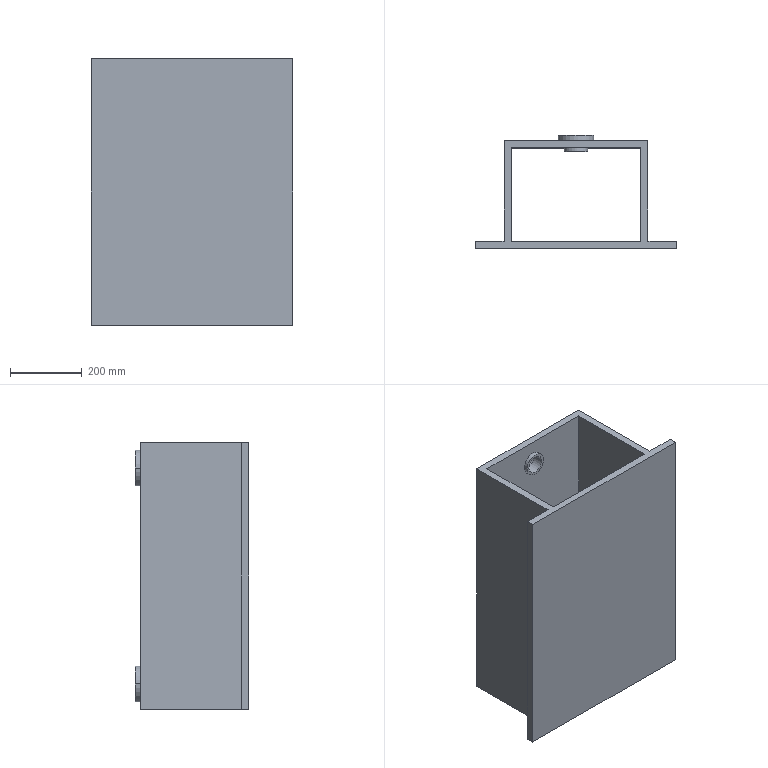Component | SolidWorks | IdlerRollerBase-1 | 5 solids | 44 faces | box 560 x 315 x 740 mm | volume 21872191 mm3 | cylinder 22 | plane 22 | commonest cylinder face diameters 50 x8 65 x8 100 x6 | material 45
build123d program:
from build123d import *

# Parameters (mm, degrees)
SKETCH1_W             = 400
SKETCH1_H             = 300
SKETCH1_W_2           = 360
SKETCH1_H_2           = 260
BOSS_EXTRUDE1_DEPTH   = 740
SKETCH3_W             = 740
SKETCH3_H             = 20
BOSS_EXTRUDE2_DEPTH   = 80
CUT_EXTRUDE1_REACH    = 848.168
SKETCH4_R             = 32.5
SKETCH5_R             = 50
SKETCH5_R_2           = 25
BOSS_EXTRUDE3_DEPTH   = 15
BOSS_EXTRUDE3_2_DEPTH = 15
SKETCH6_R             = 32.5
SKETCH6_R_2           = 25
BOSS_EXTRUDE4_DEPTH   = 30
BOSS_EXTRUDE4_2_DEPTH = 30
SKETCH7_R             = 50
CUT_EXTRUDE2_DEPTH    = 20


with BuildPart() as part:
    # Sketch1 → Boss-Extrude1 (new body)
    with BuildSketch(Plane.XY):
        Rectangle(SKETCH1_W, SKETCH1_H)
        Rectangle(SKETCH1_W_2, SKETCH1_H_2, mode=Mode.SUBTRACT)
    extrude(amount=BOSS_EXTRUDE1_DEPTH)

    # Sketch3 → Boss-Extrude2 (add)
    with BuildSketch(Plane(origin=(200, 0, 0), x_dir=(0, 0, -1), z_dir=(1, 0, 0))):
        with Locations((-370, -140)):
            Rectangle(SKETCH3_W, SKETCH3_H)
    boss_extrude2 = extrude(amount=BOSS_EXTRUDE2_DEPTH)

    # Mirror1: Boss-Extrude2 across plane
    add(boss_extrude2.mirror(Plane(origin=(0, 0, 0), x_dir=(0, 0, 1), z_dir=(1, 0, 0))))

    # Sketch4 → Cut-Extrude1 (cut, up to next)
    with BuildSketch(Plane(origin=(0, 150, 0), x_dir=(1, 0, 0), z_dir=(0, 1, 0)), mode=Mode.PRIVATE) as cut_extrude1_sk1:
        with Locations(Location((0, -670, 0), (0, 0, 180))):
            Circle(SKETCH4_R)
    cut_extrude1_tool1 = extrude(cut_extrude1_sk1.sketch, amount=-CUT_EXTRUDE1_REACH, mode=Mode.PRIVATE) & part.part
    # Sketch4 → Cut-Extrude1 (cut, up to next)
    with BuildSketch(Plane(origin=(0, 150, 0), x_dir=(1, 0, 0), z_dir=(0, 1, 0)), mode=Mode.PRIVATE) as cut_extrude1_sk2:
        with Locations(Location((0, -70, 0), (0, 0, 180))):
            Circle(SKETCH4_R)
    cut_extrude1_tool2 = extrude(cut_extrude1_sk2.sketch, amount=-CUT_EXTRUDE1_REACH, mode=Mode.PRIVATE) & part.part
    add(cut_extrude1_tool1.solids().sort_by_distance((0, 150, 670))[0], mode=Mode.SUBTRACT)
    add(cut_extrude1_tool2.solids().sort_by_distance((0, 150, 70))[0], mode=Mode.SUBTRACT)

    # Sketch7 → Cut-Extrude2 (cut)
    with BuildSketch(Plane(origin=(0, 150, 0), x_dir=(1, 0, 0), z_dir=(0, 1, 0))):
        with Locations(Location((0, -370, 0), (0, 0, 180))):
            Circle(SKETCH7_R)
    extrude(amount=-CUT_EXTRUDE2_DEPTH, mode=Mode.SUBTRACT)


with BuildPart() as body_2:
    # Sketch5 → Boss-Extrude3 (new body)
    with BuildSketch(Plane(origin=(0, 150, 0), x_dir=(1, 0, 0), z_dir=(0, 1, 0))):
        with Locations(Location((0, -670, 0), (0, 0, 180))):
            Circle(SKETCH5_R)
        with Locations(Location((0, -670, 0), (0, 0, 180))):
            Circle(SKETCH5_R_2, mode=Mode.SUBTRACT)
    extrude(amount=BOSS_EXTRUDE3_DEPTH)


with BuildPart() as body_3:
    # Sketch5 → Boss-Extrude3 2 (new body)
    with BuildSketch(Plane(origin=(0, 150, 0), x_dir=(1, 0, 0), z_dir=(0, 1, 0))):
        with Locations(Location((0, -70, 0), (0, 0, 180))):
            Circle(SKETCH5_R)
        with Locations(Location((0, -70, 0), (0, 0, 180))):
            Circle(SKETCH5_R_2, mode=Mode.SUBTRACT)
    extrude(amount=BOSS_EXTRUDE3_2_DEPTH)


with BuildPart() as body_4:
    # Sketch6 → Boss-Extrude4 (new body)
    with BuildSketch(Plane.XZ.offset(-150)):
        with Locations((0, 670)):
            Circle(SKETCH6_R)
        with Locations((0, 670)):
            Circle(SKETCH6_R_2, mode=Mode.SUBTRACT)
    extrude(amount=BOSS_EXTRUDE4_DEPTH)


with BuildPart() as body_5:
    # Sketch6 → Boss-Extrude4 2 (new body)
    with BuildSketch(Plane.XZ.offset(-150)):
        with Locations((0, 70)):
            Circle(SKETCH6_R)
        with Locations((0, 70)):
            Circle(SKETCH6_R_2, mode=Mode.SUBTRACT)
    extrude(amount=BOSS_EXTRUDE4_2_DEPTH)


solid = Compound([part.part, body_2.part, body_3.part, body_4.part, body_5.part])

# Placed as in the assembly
solid = solid.moved(Location((-90.813, -261.571, -270), (0, 0, 0)))